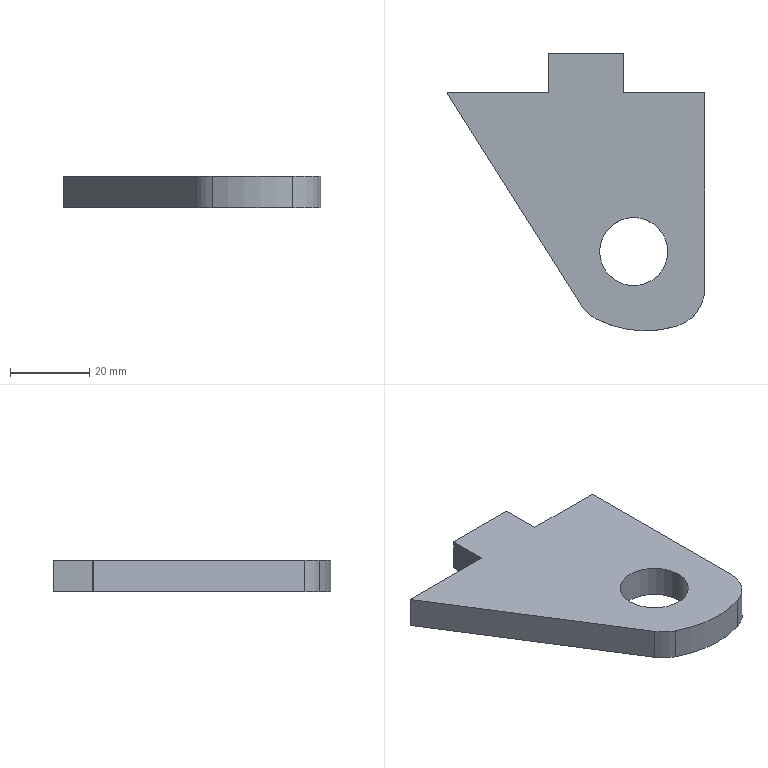Component | SolidWorks | SteeringLug-1 | 1 solid | 15 faces | box 65 x 70.05 x 8 mm | volume 21448 mm3 | plane 10 | cylinder 5 | commonest cylinder face diameters 17.2 x2 20 x2 54.376 x1 | material Q235
build123d program:
from build123d import *

# Parameters (mm, degrees)
SKETCH1_R           = 8.6
BOSS_EXTRUDE1_DEPTH = 8


with BuildPart() as part:
    # Sketch1 → Boss-Extrude1 (new body)
    with BuildSketch(Plane.XY):
        with BuildLine():
            Line((-20.075, 21.524), (-20.075, -8.476))
            Line((-20.075, -8.476), (-20.075, -18.476))
            Line((-20.075, -18.476), (-20.075, -18.557))
            Line((-20.075, -18.557), (0.3731, -18.557))
            Line((0.3731, -18.557), (0.3731, -28.557))
            Line((0.3731, -28.557), (19.373, -28.557))
            Line((19.373, -28.557), (19.373, -18.557))
            Line((19.373, -18.557), (30.873, -18.557))
            Line((30.873, -18.557), (31.373, -18.557))
            Line((31.373, -18.557), (44.925, -18.557))
            Line((44.925, -18.557), (44.925, -18.476))
            Line((44.925, -18.476), (11.211, 34.948))
            ThreePointArc((11.211, 34.948), (9.5, 36.993), (7.309, 38.513))
            ThreePointArc((7.309, 38.513), (-2.661, 41.39), (-12.984, 40.321))
            ThreePointArc((-12.984, 40.321), (-18.109, 36.708), (-20.075, 30.754))
            Line((-20.075, 30.754), (-20.075, 21.524))
        make_face()
        with Locations((-2.127, 21.524)):
            Circle(SKETCH1_R, mode=Mode.SUBTRACT)
    extrude(amount=BOSS_EXTRUDE1_DEPTH)


solid = part.part

# Placed as in the assembly
solid = solid.moved(Location((-807.646, 1758.917, 2678.363), (0, 0, 180)))
STEP:
#1=COLOUR_RGB('',0.7922,0.8196,0.9333);
#2=FILL_AREA_STYLE_COLOUR('',#1);
#3=FILL_AREA_STYLE('',(#2));
#4=SURFACE_STYLE_FILL_AREA(#3);
#5=SURFACE_SIDE_STYLE('',(#4));
#6=SURFACE_STYLE_USAGE(.BOTH.,#5);
#7=PRESENTATION_STYLE_ASSIGNMENT((#6));
#8=CARTESIAN_POINT('',(-31.375,68.401,105.762));
#9=VERTEX_POINT('',#8);
#10=CARTESIAN_POINT('',(-32.052,68.401,105.762));
#11=VERTEX_POINT('',#10);
#12=CARTESIAN_POINT('',(-31.713,68.401,105.762));
#13=DIRECTION('',(-0.,0.,1.));
#14=DIRECTION('',(-1.,0.,0.));
#15=AXIS2_PLACEMENT_3D('',#12,#13,#14);
#16=CIRCLE('',#15,0.3386);
#17=EDGE_CURVE('',#9,#11,#16,.T.);
#18=ORIENTED_EDGE('',*,*,#17,.T.);
#19=CARTESIAN_POINT('',(-32.052,68.401,105.447));
#20=VERTEX_POINT('',#19);
#21=CARTESIAN_POINT('',(-32.052,68.401,105.762));
#22=DIRECTION('',(0.,-0.,-1.));
#23=VECTOR('',#22,39.37);
#24=LINE('',#21,#23);
#25=EDGE_CURVE('',#11,#20,#24,.T.);
#26=ORIENTED_EDGE('',*,*,#25,.T.);
#27=CARTESIAN_POINT('',(-31.375,68.401,105.447));
#28=VERTEX_POINT('',#27);
#29=CARTESIAN_POINT('',(-31.713,68.401,105.447));
#30=DIRECTION('',(-0.,0.,1.));
#31=DIRECTION('',(-1.,0.,0.));
#32=AXIS2_PLACEMENT_3D('',#29,#30,#31);
#33=CIRCLE('',#32,0.3386);
#34=EDGE_CURVE('',#28,#20,#33,.T.);
#35=ORIENTED_EDGE('',*,*,#34,.F.);
#36=CARTESIAN_POINT('',(-31.375,68.401,105.762));
#37=DIRECTION('',(0.,-0.,-1.));
#38=VECTOR('',#37,39.37);
#39=LINE('',#36,#38);
#40=EDGE_CURVE('',#9,#28,#39,.T.);
#41=ORIENTED_EDGE('',*,*,#40,.F.);
#42=EDGE_LOOP('',(#18,#26,#35,#41));
#43=FACE_OUTER_BOUND('',#42,.T.);
#44=CARTESIAN_POINT('',(-31.713,68.401,105.762));
#45=DIRECTION('',(0.,-0.,-1.));
#46=DIRECTION('',(1.,0.,0.));
#47=AXIS2_PLACEMENT_3D('',#44,#45,#46);
#48=CYLINDRICAL_SURFACE('',#47,0.3386);
#49=ADVANCED_FACE('',(#43),#48,.F.);
#50=CARTESIAN_POINT('',(-32.238,67.873,105.762));
#51=VERTEX_POINT('',#50);
#52=CARTESIAN_POINT('',(-32.085,67.732,105.762));
#53=VERTEX_POINT('',#52);
#54=CARTESIAN_POINT('',(-31.906,68.083,105.762));
#55=DIRECTION('',(-0.,0.,1.));
#56=DIRECTION('',(-1.,0.,0.));
#57=AXIS2_PLACEMENT_3D('',#54,#55,#56);
#58=CIRCLE('',#57,0.3937);
#59=EDGE_CURVE('',#51,#53,#58,.T.);
#60=ORIENTED_EDGE('',*,*,#59,.T.);
#61=CARTESIAN_POINT('',(-31.286,67.661,105.762));
#62=VERTEX_POINT('',#61);
#63=CARTESIAN_POINT('',(-31.597,68.685,105.762));
#64=DIRECTION('',(-0.,0.,1.));
#65=DIRECTION('',(-1.,0.,0.));
#66=AXIS2_PLACEMENT_3D('',#63,#64,#65);
#67=CIRCLE('',#66,1.07);
#68=EDGE_CURVE('',#53,#62,#67,.T.);
#69=ORIENTED_EDGE('',*,*,#68,.T.);
#70=CARTESIAN_POINT('',(-31.007,68.038,105.762));
#71=VERTEX_POINT('',#70);
#72=CARTESIAN_POINT('',(-31.4,68.038,105.762));
#73=DIRECTION('',(-0.,0.,1.));
#74=DIRECTION('',(-1.,0.,0.));
#75=AXIS2_PLACEMENT_3D('',#72,#73,#74);
#76=CIRCLE('',#75,0.3937);
#77=EDGE_CURVE('',#62,#71,#76,.T.);
#78=ORIENTED_EDGE('',*,*,#77,.T.);
#79=CARTESIAN_POINT('',(-31.007,69.979,105.762));
#80=VERTEX_POINT('',#79);
#81=CARTESIAN_POINT('',(-31.007,68.038,105.762));
#82=DIRECTION('',(0.,1.,-0.));
#83=VECTOR('',#82,39.37);
#84=LINE('',#81,#83);
#85=EDGE_CURVE('',#71,#80,#84,.T.);
#86=ORIENTED_EDGE('',*,*,#85,.T.);
#87=CARTESIAN_POINT('',(-31.812,69.979,105.762));
#88=VERTEX_POINT('',#87);
#89=CARTESIAN_POINT('',(-31.812,69.979,105.762));
#90=DIRECTION('',(-1.,-0.,-0.));
#91=VECTOR('',#90,39.37);
#92=LINE('',#89,#91);
#93=EDGE_CURVE('',#80,#88,#92,.T.);
#94=ORIENTED_EDGE('',*,*,#93,.T.);
#95=CARTESIAN_POINT('',(-31.812,70.373,105.762));
#96=VERTEX_POINT('',#95);
#97=CARTESIAN_POINT('',(-31.812,69.979,105.762));
#98=DIRECTION('',(-0.,1.,-0.));
#99=VECTOR('',#98,39.37);
#100=LINE('',#97,#99);
#101=EDGE_CURVE('',#88,#96,#100,.T.);
#102=ORIENTED_EDGE('',*,*,#101,.T.);
#103=CARTESIAN_POINT('',(-32.56,70.373,105.762));
#104=VERTEX_POINT('',#103);
#105=CARTESIAN_POINT('',(-31.812,70.373,105.762));
#106=DIRECTION('',(-1.,-0.,-0.));
#107=VECTOR('',#106,39.37);
#108=LINE('',#105,#107);
#109=EDGE_CURVE('',#96,#104,#108,.T.);
#110=ORIENTED_EDGE('',*,*,#109,.T.);
#111=CARTESIAN_POINT('',(-32.56,69.979,105.762));
#112=VERTEX_POINT('',#111);
#113=CARTESIAN_POINT('',(-32.56,70.373,105.762));
#114=DIRECTION('',(0.,-1.,0.));
#115=VECTOR('',#114,39.37);
#116=LINE('',#113,#115);
#117=EDGE_CURVE('',#104,#112,#116,.T.);
#118=ORIENTED_EDGE('',*,*,#117,.T.);
#119=CARTESIAN_POINT('',(-33.566,69.979,105.762));
#120=VERTEX_POINT('',#119);
#121=CARTESIAN_POINT('',(-32.56,69.979,105.762));
#122=DIRECTION('',(-1.,-0.,-0.));
#123=VECTOR('',#122,39.37);
#124=LINE('',#121,#123);
#125=EDGE_CURVE('',#112,#120,#124,.T.);
#126=ORIENTED_EDGE('',*,*,#125,.T.);
#127=CARTESIAN_POINT('',(-33.566,69.976,105.762));
#128=VERTEX_POINT('',#127);
#129=CARTESIAN_POINT('',(-33.566,69.979,105.762));
#130=DIRECTION('',(0.,-1.,0.));
#131=VECTOR('',#130,39.37);
#132=LINE('',#129,#131);
#133=EDGE_CURVE('',#120,#128,#132,.T.);
#134=ORIENTED_EDGE('',*,*,#133,.T.);
#135=CARTESIAN_POINT('',(-33.566,69.976,105.762));
#136=DIRECTION('',(0.5337,-0.8457,0.));
#137=VECTOR('',#136,39.37);
#138=LINE('',#135,#137);
#139=EDGE_CURVE('',#128,#51,#138,.T.);
#140=ORIENTED_EDGE('',*,*,#139,.T.);
#141=EDGE_LOOP('',(#60,#69,#78,#86,#94,#102,#110,#118,#126,#134,#140));
#142=FACE_OUTER_BOUND('',#141,.T.);
#143=ORIENTED_EDGE('',*,*,#17,.F.);
#144=CARTESIAN_POINT('',(-31.713,68.401,105.762));
#145=DIRECTION('',(-0.,0.,1.));
#146=DIRECTION('',(-1.,0.,0.));
#147=AXIS2_PLACEMENT_3D('',#144,#145,#146);
#148=CIRCLE('',#147,0.3386);
#149=EDGE_CURVE('',#11,#9,#148,.T.);
#150=ORIENTED_EDGE('',*,*,#149,.F.);
#151=EDGE_LOOP('',(#143,#150));
#152=FACE_BOUND('',#151,.T.);
#153=CARTESIAN_POINT('',(-31.906,68.083,105.762));
#154=DIRECTION('',(-0.,0.,1.));
#155=DIRECTION('',(-1.,-0.,-0.));
#156=AXIS2_PLACEMENT_3D('',#153,#154,#155);
#157=PLANE('',#156);
#158=ADVANCED_FACE('',(#142,#152),#157,.T.);
#159=CARTESIAN_POINT('',(-32.238,67.873,105.447));
#160=VERTEX_POINT('',#159);
#161=CARTESIAN_POINT('',(-32.085,67.732,105.447));
#162=VERTEX_POINT('',#161);
#163=CARTESIAN_POINT('',(-31.906,68.083,105.447));
#164=DIRECTION('',(-0.,0.,1.));
#165=DIRECTION('',(-1.,0.,0.));
#166=AXIS2_PLACEMENT_3D('',#163,#164,#165);
#167=CIRCLE('',#166,0.3937);
#168=EDGE_CURVE('',#160,#162,#167,.T.);
#169=ORIENTED_EDGE('',*,*,#168,.F.);
#170=CARTESIAN_POINT('',(-33.566,69.976,105.447));
#171=VERTEX_POINT('',#170);
#172=CARTESIAN_POINT('',(-33.566,69.976,105.447));
#173=DIRECTION('',(0.5337,-0.8457,0.));
#174=VECTOR('',#173,39.37);
#175=LINE('',#172,#174);
#176=EDGE_CURVE('',#171,#160,#175,.T.);
#177=ORIENTED_EDGE('',*,*,#176,.F.);
#178=CARTESIAN_POINT('',(-33.566,69.979,105.447));
#179=VERTEX_POINT('',#178);
#180=CARTESIAN_POINT('',(-33.566,69.979,105.447));
#181=DIRECTION('',(0.,-1.,0.));
#182=VECTOR('',#181,39.37);
#183=LINE('',#180,#182);
#184=EDGE_CURVE('',#179,#171,#183,.T.);
#185=ORIENTED_EDGE('',*,*,#184,.F.);
#186=CARTESIAN_POINT('',(-32.56,69.979,105.447));
#187=VERTEX_POINT('',#186);
#188=CARTESIAN_POINT('',(-33.032,69.979,105.447));
#189=DIRECTION('',(-1.,-0.,-0.));
#190=VECTOR('',#189,39.37);
#191=LINE('',#188,#190);
#192=EDGE_CURVE('',#187,#179,#191,.T.);
#193=ORIENTED_EDGE('',*,*,#192,.F.);
#194=CARTESIAN_POINT('',(-32.56,70.373,105.447));
#195=VERTEX_POINT('',#194);
#196=CARTESIAN_POINT('',(-32.56,70.373,105.447));
#197=DIRECTION('',(0.,-1.,0.));
#198=VECTOR('',#197,39.37);
#199=LINE('',#196,#198);
#200=EDGE_CURVE('',#195,#187,#199,.T.);
#201=ORIENTED_EDGE('',*,*,#200,.F.);
#202=CARTESIAN_POINT('',(-31.812,70.373,105.447));
#203=VERTEX_POINT('',#202);
#204=CARTESIAN_POINT('',(-31.812,70.373,105.447));
#205=DIRECTION('',(-1.,-0.,-0.));
#206=VECTOR('',#205,39.37);
#207=LINE('',#204,#206);
#208=EDGE_CURVE('',#203,#195,#207,.T.);
#209=ORIENTED_EDGE('',*,*,#208,.F.);
#210=CARTESIAN_POINT('',(-31.812,69.979,105.447));
#211=VERTEX_POINT('',#210);
#212=CARTESIAN_POINT('',(-31.812,69.979,105.447));
#213=DIRECTION('',(-0.,1.,-0.));
#214=VECTOR('',#213,39.37);
#215=LINE('',#212,#214);
#216=EDGE_CURVE('',#211,#203,#215,.T.);
#217=ORIENTED_EDGE('',*,*,#216,.F.);
#218=CARTESIAN_POINT('',(-31.007,69.979,105.447));
#219=VERTEX_POINT('',#218);
#220=CARTESIAN_POINT('',(-31.812,69.979,105.447));
#221=DIRECTION('',(-1.,-0.,-0.));
#222=VECTOR('',#221,39.37);
#223=LINE('',#220,#222);
#224=EDGE_CURVE('',#219,#211,#223,.T.);
#225=ORIENTED_EDGE('',*,*,#224,.F.);
#226=CARTESIAN_POINT('',(-31.007,68.038,105.447));
#227=VERTEX_POINT('',#226);
#228=CARTESIAN_POINT('',(-31.007,69.979,105.447));
#229=DIRECTION('',(-0.,1.,-0.));
#230=VECTOR('',#229,39.37);
#231=LINE('',#228,#230);
#232=EDGE_CURVE('',#227,#219,#231,.T.);
#233=ORIENTED_EDGE('',*,*,#232,.F.);
#234=CARTESIAN_POINT('',(-31.286,67.661,105.447));
#235=VERTEX_POINT('',#234);
#236=CARTESIAN_POINT('',(-31.4,68.038,105.447));
#237=DIRECTION('',(-0.,0.,1.));
#238=DIRECTION('',(-1.,0.,0.));
#239=AXIS2_PLACEMENT_3D('',#236,#237,#238);
#240=CIRCLE('',#239,0.3937);
#241=EDGE_CURVE('',#235,#227,#240,.T.);
#242=ORIENTED_EDGE('',*,*,#241,.F.);
#243=CARTESIAN_POINT('',(-31.597,68.685,105.447));
#244=DIRECTION('',(-0.,0.,1.));
#245=DIRECTION('',(-1.,0.,0.));
#246=AXIS2_PLACEMENT_3D('',#243,#244,#245);
#247=CIRCLE('',#246,1.07);
#248=EDGE_CURVE('',#162,#235,#247,.T.);
#249=ORIENTED_EDGE('',*,*,#248,.F.);
#250=EDGE_LOOP('',(#169,#177,#185,#193,#201,#209,#217,#225,#233,#242,#249));
#251=FACE_OUTER_BOUND('',#250,.T.);
#252=ORIENTED_EDGE('',*,*,#34,.T.);
#253=CARTESIAN_POINT('',(-31.713,68.401,105.447));
#254=DIRECTION('',(-0.,0.,1.));
#255=DIRECTION('',(-1.,0.,0.));
#256=AXIS2_PLACEMENT_3D('',#253,#254,#255);
#257=CIRCLE('',#256,0.3386);
#258=EDGE_CURVE('',#20,#28,#257,.T.);
#259=ORIENTED_EDGE('',*,*,#258,.T.);
#260=EDGE_LOOP('',(#252,#259));
#261=FACE_BOUND('',#260,.T.);
#262=CARTESIAN_POINT('',(-31.906,68.083,105.447));
#263=DIRECTION('',(-0.,0.,1.));
#264=DIRECTION('',(-1.,-0.,-0.));
#265=AXIS2_PLACEMENT_3D('',#262,#263,#264);
#266=PLANE('',#265);
#267=ADVANCED_FACE('',(#251,#261),#266,.F.);
#268=ORIENTED_EDGE('',*,*,#168,.T.);
#269=CARTESIAN_POINT('',(-32.085,67.732,105.762));
#270=DIRECTION('',(0.,-0.,-1.));
#271=VECTOR('',#270,39.37);
#272=LINE('',#269,#271);
#273=EDGE_CURVE('',#53,#162,#272,.T.);
#274=ORIENTED_EDGE('',*,*,#273,.F.);
#275=ORIENTED_EDGE('',*,*,#59,.F.);
#276=CARTESIAN_POINT('',(-32.238,67.873,105.762));
#277=DIRECTION('',(0.,-0.,-1.));
#278=VECTOR('',#277,39.37);
#279=LINE('',#276,#278);
#280=EDGE_CURVE('',#51,#160,#279,.T.);
#281=ORIENTED_EDGE('',*,*,#280,.T.);
#282=EDGE_LOOP('',(#268,#274,#275,#281));
#283=FACE_OUTER_BOUND('',#282,.T.);
#284=CARTESIAN_POINT('',(-31.906,68.083,105.762));
#285=DIRECTION('',(0.,-0.,-1.));
#286=DIRECTION('',(1.,0.,0.));
#287=AXIS2_PLACEMENT_3D('',#284,#285,#286);
#288=CYLINDRICAL_SURFACE('',#287,0.3937);
#289=ADVANCED_FACE('',(#283),#288,.T.);
#290=ORIENTED_EDGE('',*,*,#248,.T.);
#291=CARTESIAN_POINT('',(-31.286,67.661,105.762));
#292=DIRECTION('',(0.,-0.,-1.));
#293=VECTOR('',#292,39.37);
#294=LINE('',#291,#293);
#295=EDGE_CURVE('',#62,#235,#294,.T.);
#296=ORIENTED_EDGE('',*,*,#295,.F.);
#297=ORIENTED_EDGE('',*,*,#68,.F.);
#298=ORIENTED_EDGE('',*,*,#273,.T.);
#299=EDGE_LOOP('',(#290,#296,#297,#298));
#300=FACE_OUTER_BOUND('',#299,.T.);
#301=CARTESIAN_POINT('',(-31.597,68.685,105.762));
#302=DIRECTION('',(0.,-0.,-1.));
#303=DIRECTION('',(1.,0.,0.));
#304=AXIS2_PLACEMENT_3D('',#301,#302,#303);
#305=CYLINDRICAL_SURFACE('',#304,1.07);
#306=ADVANCED_FACE('',(#300),#305,.T.);
#307=ORIENTED_EDGE('',*,*,#241,.T.);
#308=CARTESIAN_POINT('',(-31.007,68.038,105.762));
#309=DIRECTION('',(0.,-0.,-1.));
#310=VECTOR('',#309,39.37);
#311=LINE('',#308,#310);
#312=EDGE_CURVE('',#71,#227,#311,.T.);
#313=ORIENTED_EDGE('',*,*,#312,.F.);
#314=ORIENTED_EDGE('',*,*,#77,.F.);
#315=ORIENTED_EDGE('',*,*,#295,.T.);
#316=EDGE_LOOP('',(#307,#313,#314,#315));
#317=FACE_OUTER_BOUND('',#316,.T.);
#318=CARTESIAN_POINT('',(-31.4,68.038,105.762));
#319=DIRECTION('',(0.,-0.,-1.));
#320=DIRECTION('',(1.,0.,0.));
#321=AXIS2_PLACEMENT_3D('',#318,#319,#320);
#322=CYLINDRICAL_SURFACE('',#321,0.3937);
#323=ADVANCED_FACE('',(#317),#322,.T.);
#324=ORIENTED_EDGE('',*,*,#232,.T.);
#325=CARTESIAN_POINT('',(-31.007,69.979,105.762));
#326=DIRECTION('',(0.,-0.,-1.));
#327=VECTOR('',#326,39.37);
#328=LINE('',#325,#327);
#329=EDGE_CURVE('',#80,#219,#328,.T.);
#330=ORIENTED_EDGE('',*,*,#329,.F.);
#331=ORIENTED_EDGE('',*,*,#85,.F.);
#332=ORIENTED_EDGE('',*,*,#312,.T.);
#333=EDGE_LOOP('',(#324,#330,#331,#332));
#334=FACE_OUTER_BOUND('',#333,.T.);
#335=CARTESIAN_POINT('',(-31.007,69.979,105.762));
#336=DIRECTION('',(-1.,-0.,-0.));
#337=DIRECTION('',(0.,-0.,-1.));
#338=AXIS2_PLACEMENT_3D('',#335,#336,#337);
#339=PLANE('',#338);
#340=ADVANCED_FACE('',(#334),#339,.F.);
#341=ORIENTED_EDGE('',*,*,#224,.T.);
#342=CARTESIAN_POINT('',(-31.812,69.979,105.762));
#343=DIRECTION('',(0.,-0.,-1.));
#344=VECTOR('',#343,39.37);
#345=LINE('',#342,#344);
#346=EDGE_CURVE('',#88,#211,#345,.T.);
#347=ORIENTED_EDGE('',*,*,#346,.F.);
#348=ORIENTED_EDGE('',*,*,#93,.F.);
#349=ORIENTED_EDGE('',*,*,#329,.T.);
#350=EDGE_LOOP('',(#341,#347,#348,#349));
#351=FACE_OUTER_BOUND('',#350,.T.);
#352=CARTESIAN_POINT('',(-31.812,69.979,105.762));
#353=DIRECTION('',(0.,-1.,0.));
#354=DIRECTION('',(-0.,0.,1.));
#355=AXIS2_PLACEMENT_3D('',#352,#353,#354);
#356=PLANE('',#355);
#357=ADVANCED_FACE('',(#351),#356,.F.);
#358=ORIENTED_EDGE('',*,*,#216,.T.);
#359=CARTESIAN_POINT('',(-31.812,70.373,105.762));
#360=DIRECTION('',(0.,-0.,-1.));
#361=VECTOR('',#360,39.37);
#362=LINE('',#359,#361);
#363=EDGE_CURVE('',#96,#203,#362,.T.);
#364=ORIENTED_EDGE('',*,*,#363,.F.);
#365=ORIENTED_EDGE('',*,*,#101,.F.);
#366=ORIENTED_EDGE('',*,*,#346,.T.);
#367=EDGE_LOOP('',(#358,#364,#365,#366));
#368=FACE_OUTER_BOUND('',#367,.T.);
#369=CARTESIAN_POINT('',(-31.812,69.979,105.762));
#370=DIRECTION('',(-1.,-0.,-0.));
#371=DIRECTION('',(0.,-0.,-1.));
#372=AXIS2_PLACEMENT_3D('',#369,#370,#371);
#373=PLANE('',#372);
#374=ADVANCED_FACE('',(#368),#373,.F.);
#375=ORIENTED_EDGE('',*,*,#208,.T.);
#376=CARTESIAN_POINT('',(-32.56,70.373,105.762));
#377=DIRECTION('',(0.,-0.,-1.));
#378=VECTOR('',#377,39.37);
#379=LINE('',#376,#378);
#380=EDGE_CURVE('',#104,#195,#379,.T.);
#381=ORIENTED_EDGE('',*,*,#380,.F.);
#382=ORIENTED_EDGE('',*,*,#109,.F.);
#383=ORIENTED_EDGE('',*,*,#363,.T.);
#384=EDGE_LOOP('',(#375,#381,#382,#383));
#385=FACE_OUTER_BOUND('',#384,.T.);
#386=CARTESIAN_POINT('',(-31.812,70.373,105.762));
#387=DIRECTION('',(0.,-1.,0.));
#388=DIRECTION('',(-0.,0.,1.));
#389=AXIS2_PLACEMENT_3D('',#386,#387,#388);
#390=PLANE('',#389);
#391=ADVANCED_FACE('',(#385),#390,.F.);
#392=ORIENTED_EDGE('',*,*,#200,.T.);
#393=CARTESIAN_POINT('',(-32.56,69.979,105.762));
#394=DIRECTION('',(0.,-0.,-1.));
#395=VECTOR('',#394,39.37);
#396=LINE('',#393,#395);
#397=EDGE_CURVE('',#112,#187,#396,.T.);
#398=ORIENTED_EDGE('',*,*,#397,.F.);
#399=ORIENTED_EDGE('',*,*,#117,.F.);
#400=ORIENTED_EDGE('',*,*,#380,.T.);
#401=EDGE_LOOP('',(#392,#398,#399,#400));
#402=FACE_OUTER_BOUND('',#401,.T.);
#403=CARTESIAN_POINT('',(-32.56,70.373,105.762));
#404=DIRECTION('',(1.,0.,0.));
#405=DIRECTION('',(-0.,0.,1.));
#406=AXIS2_PLACEMENT_3D('',#403,#404,#405);
#407=PLANE('',#406);
#408=ADVANCED_FACE('',(#402),#407,.F.);
#409=ORIENTED_EDGE('',*,*,#192,.T.);
#410=CARTESIAN_POINT('',(-33.566,69.979,105.762));
#411=DIRECTION('',(0.,-0.,-1.));
#412=VECTOR('',#411,39.37);
#413=LINE('',#410,#412);
#414=EDGE_CURVE('',#120,#179,#413,.T.);
#415=ORIENTED_EDGE('',*,*,#414,.F.);
#416=ORIENTED_EDGE('',*,*,#125,.F.);
#417=ORIENTED_EDGE('',*,*,#397,.T.);
#418=EDGE_LOOP('',(#409,#415,#416,#417));
#419=FACE_OUTER_BOUND('',#418,.T.);
#420=CARTESIAN_POINT('',(-33.032,69.979,105.762));
#421=DIRECTION('',(0.,-1.,0.));
#422=DIRECTION('',(-0.,0.,1.));
#423=AXIS2_PLACEMENT_3D('',#420,#421,#422);
#424=PLANE('',#423);
#425=ADVANCED_FACE('',(#419),#424,.F.);
#426=ORIENTED_EDGE('',*,*,#184,.T.);
#427=CARTESIAN_POINT('',(-33.566,69.976,105.762));
#428=DIRECTION('',(0.,-0.,-1.));
#429=VECTOR('',#428,39.37);
#430=LINE('',#427,#429);
#431=EDGE_CURVE('',#128,#171,#430,.T.);
#432=ORIENTED_EDGE('',*,*,#431,.F.);
#433=ORIENTED_EDGE('',*,*,#133,.F.);
#434=ORIENTED_EDGE('',*,*,#414,.T.);
#435=EDGE_LOOP('',(#426,#432,#433,#434));
#436=FACE_OUTER_BOUND('',#435,.T.);
#437=CARTESIAN_POINT('',(-33.566,69.979,105.762));
#438=DIRECTION('',(1.,0.,0.));
#439=DIRECTION('',(-0.,1.,-0.));
#440=AXIS2_PLACEMENT_3D('',#437,#438,#439);
#441=PLANE('',#440);
#442=ADVANCED_FACE('',(#436),#441,.F.);
#443=ORIENTED_EDGE('',*,*,#176,.T.);
#444=ORIENTED_EDGE('',*,*,#280,.F.);
#445=ORIENTED_EDGE('',*,*,#139,.F.);
#446=ORIENTED_EDGE('',*,*,#431,.T.);
#447=EDGE_LOOP('',(#443,#444,#445,#446));
#448=FACE_OUTER_BOUND('',#447,.T.);
#449=CARTESIAN_POINT('',(-33.566,69.976,105.762));
#450=DIRECTION('',(0.8457,0.5337,0.));
#451=DIRECTION('',(-0.5337,0.8457,-0.));
#452=AXIS2_PLACEMENT_3D('',#449,#450,#451);
#453=PLANE('',#452);
#454=ADVANCED_FACE('',(#448),#453,.F.);
#455=ORIENTED_EDGE('',*,*,#25,.F.);
#456=ORIENTED_EDGE('',*,*,#149,.T.);
#457=ORIENTED_EDGE('',*,*,#40,.T.);
#458=ORIENTED_EDGE('',*,*,#258,.F.);
#459=EDGE_LOOP('',(#455,#456,#457,#458));
#460=FACE_OUTER_BOUND('',#459,.T.);
#461=CARTESIAN_POINT('',(-31.713,68.401,105.762));
#462=DIRECTION('',(0.,-0.,-1.));
#463=DIRECTION('',(1.,0.,0.));
#464=AXIS2_PLACEMENT_3D('',#461,#462,#463);
#465=CYLINDRICAL_SURFACE('',#464,0.3386);
#466=ADVANCED_FACE('',(#460),#465,.F.);
#467=CLOSED_SHELL('',(#49,#158,#267,#289,#306,#323,#340,#357,#374,#391,#408,#425,#442,#454,#466));
#468=MANIFOLD_SOLID_BREP('',#467);
#469=STYLED_ITEM('',(#7),#468);
#470=PRESENTATION_LAYER_ASSIGNMENT('','',(#469));
#471=(LENGTH_UNIT()NAMED_UNIT(*)SI_UNIT($,.METRE.));
#472=LENGTH_MEASURE_WITH_UNIT(LENGTH_MEASURE(0.0254),#471);
#473=DIMENSIONAL_EXPONENTS(1.,0.,0.,0.,0.,0.,0.);
#474=(CONVERSION_BASED_UNIT('',#472)LENGTH_UNIT()NAMED_UNIT(#473));
#475=UNCERTAINTY_MEASURE_WITH_UNIT(LENGTH_MEASURE(0.00001),#474,'','');
#476=(NAMED_UNIT(*)PLANE_ANGLE_UNIT()SI_UNIT($,.RADIAN.));
#477=(NAMED_UNIT(*)SI_UNIT($,.STERADIAN.)SOLID_ANGLE_UNIT());
#478=(GEOMETRIC_REPRESENTATION_CONTEXT(3)GLOBAL_UNCERTAINTY_ASSIGNED_CONTEXT((#475))GLOBAL_UNIT_ASSIGNED_CONTEXT((#474,#476,#477))REPRESENTATION_CONTEXT('',''));
#479=MECHANICAL_DESIGN_GEOMETRIC_PRESENTATION_REPRESENTATION('',(#469),#478);
#480=CARTESIAN_POINT('',(0.,0.,0.));
#481=DIRECTION('',(0.,0.,1.));
#482=DIRECTION('',(1.,0.,0.));
#483=AXIS2_PLACEMENT_3D('',#480,#481,#482);
#484=(LENGTH_UNIT()NAMED_UNIT(*)SI_UNIT($,.METRE.));
#485=LENGTH_MEASURE_WITH_UNIT(LENGTH_MEASURE(0.0254),#484);
#486=DIMENSIONAL_EXPONENTS(1.,0.,0.,0.,0.,0.,0.);
#487=(CONVERSION_BASED_UNIT('',#485)LENGTH_UNIT()NAMED_UNIT(#486));
#488=UNCERTAINTY_MEASURE_WITH_UNIT(LENGTH_MEASURE(0.00001),#487,'','');
#489=(NAMED_UNIT(*)PLANE_ANGLE_UNIT()SI_UNIT($,.RADIAN.));
#490=(NAMED_UNIT(*)SI_UNIT($,.STERADIAN.)SOLID_ANGLE_UNIT());
#491=(GEOMETRIC_REPRESENTATION_CONTEXT(3)GLOBAL_UNCERTAINTY_ASSIGNED_CONTEXT((#488))GLOBAL_UNIT_ASSIGNED_CONTEXT((#487,#489,#490))REPRESENTATION_CONTEXT('',''));
#492=ADVANCED_BREP_SHAPE_REPRESENTATION('',(#468,#483),#491);